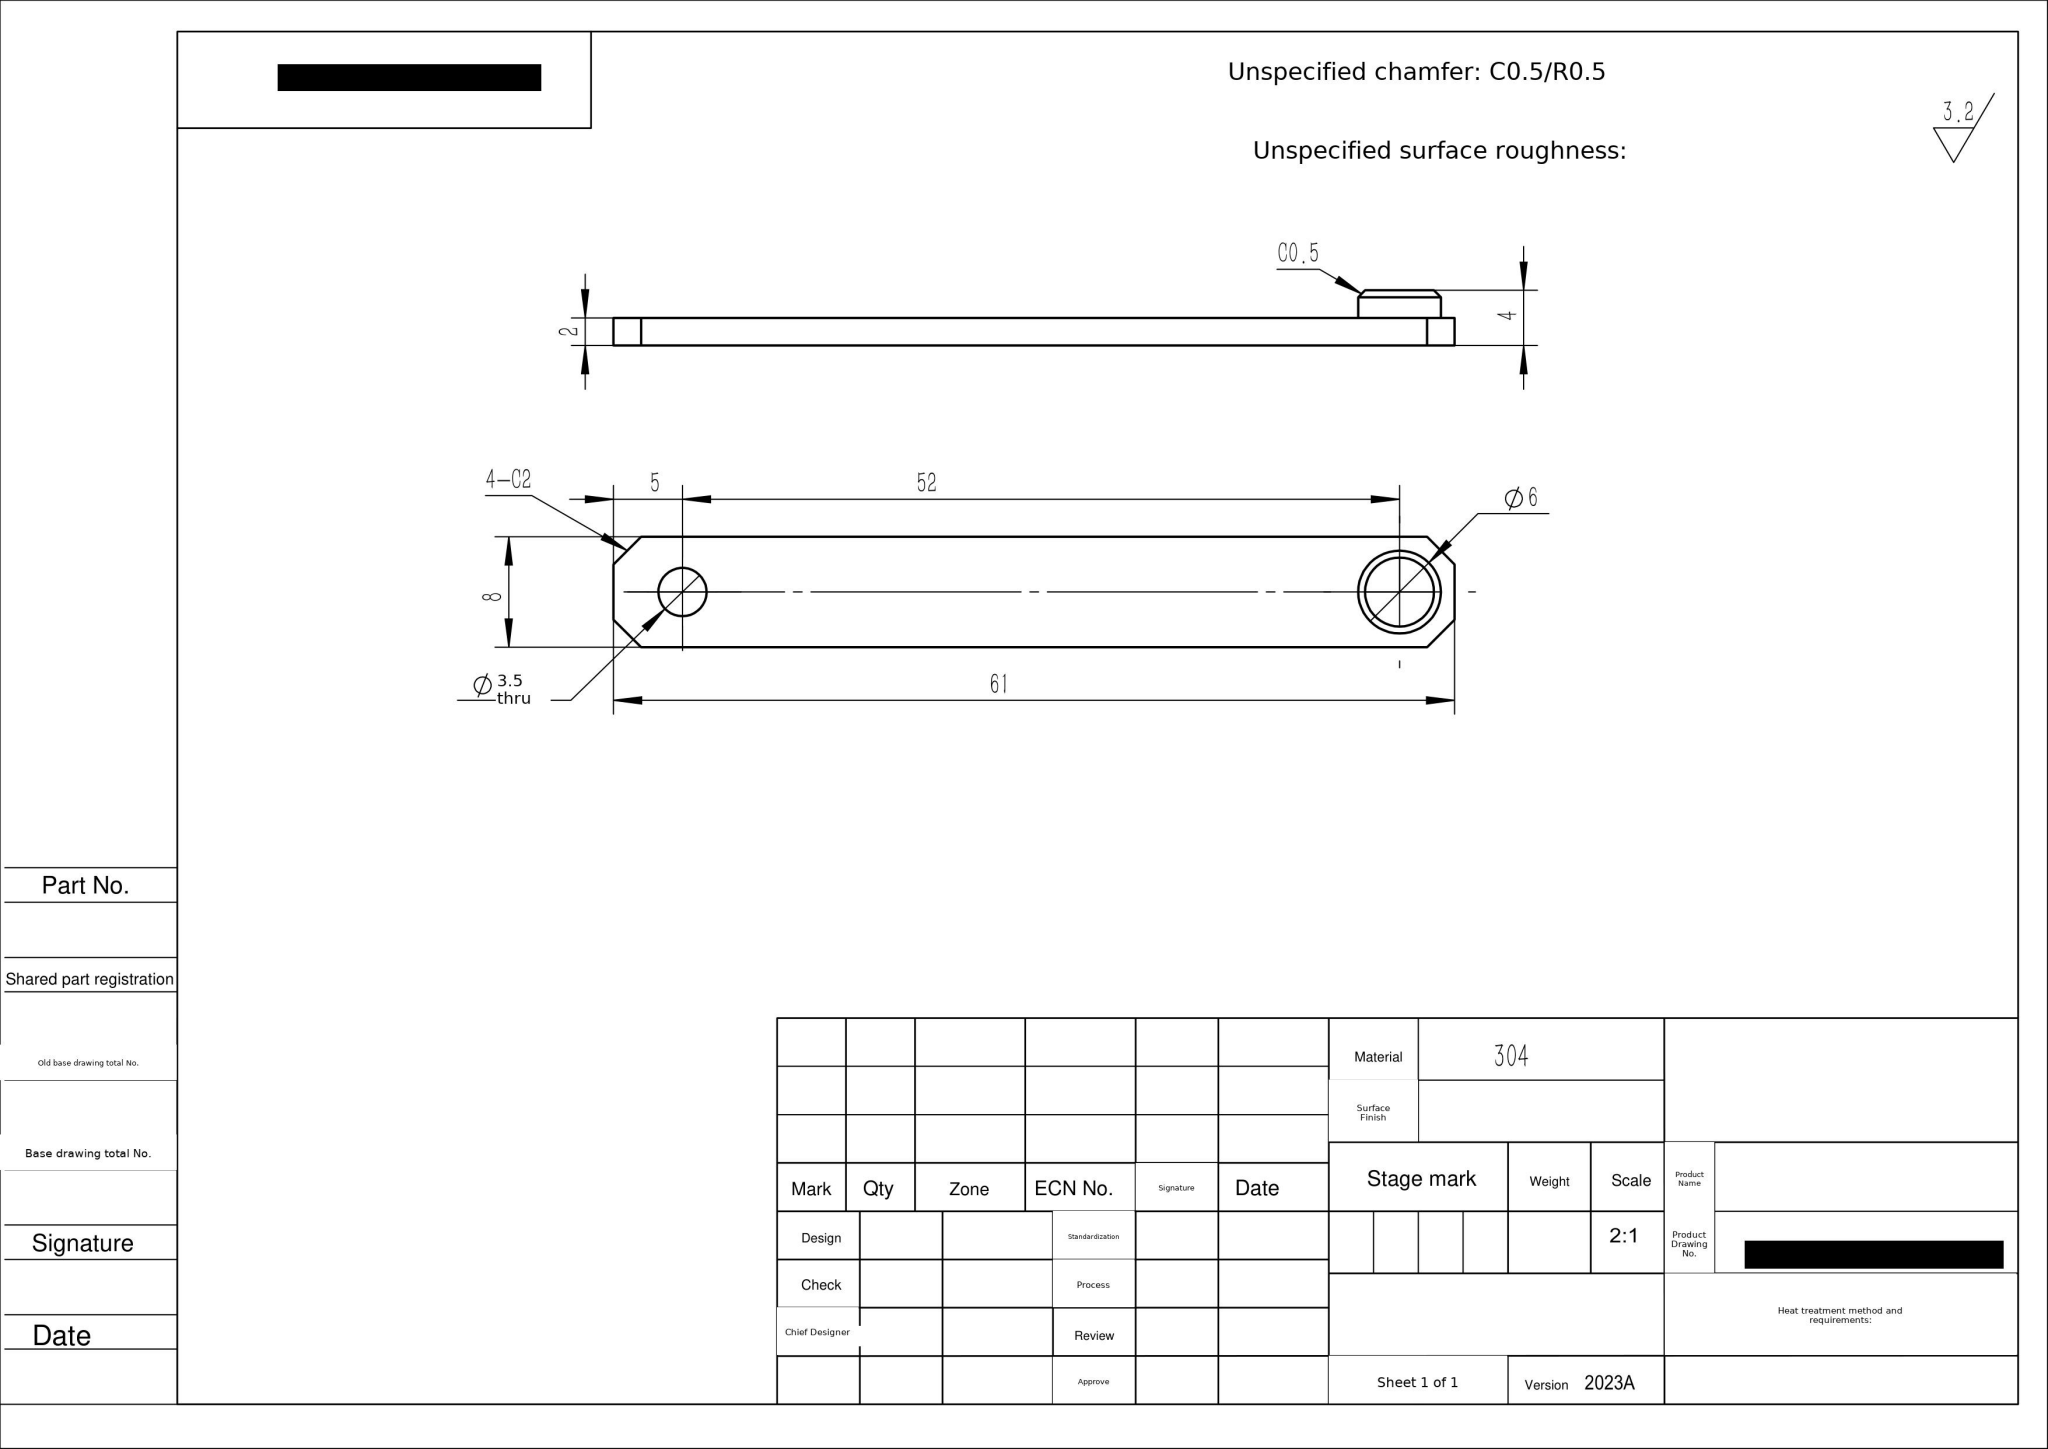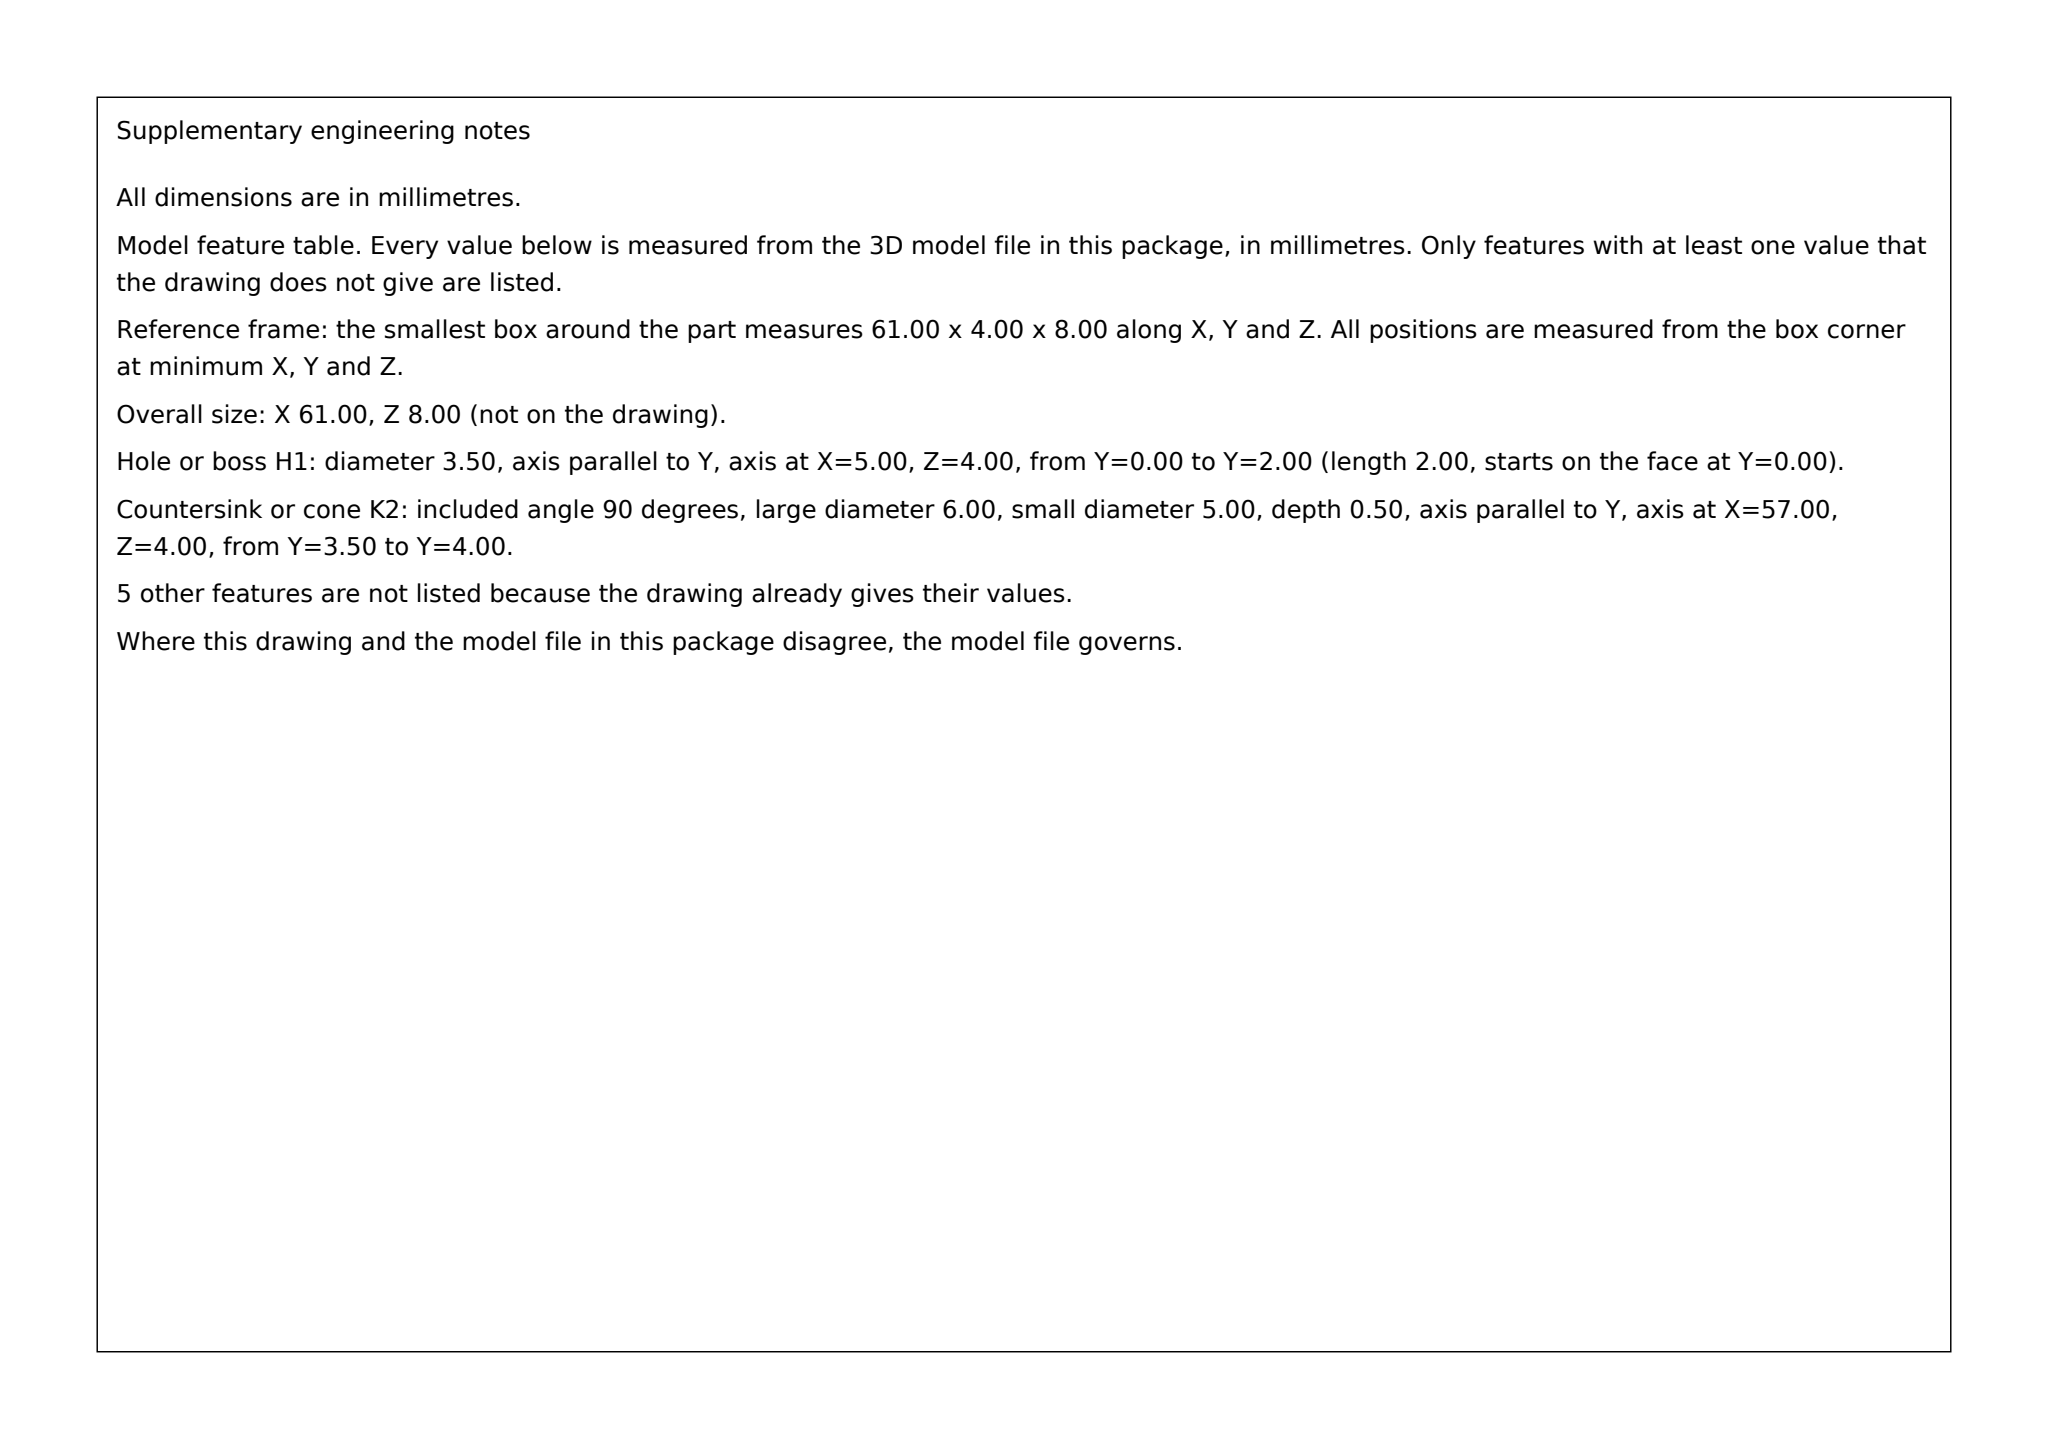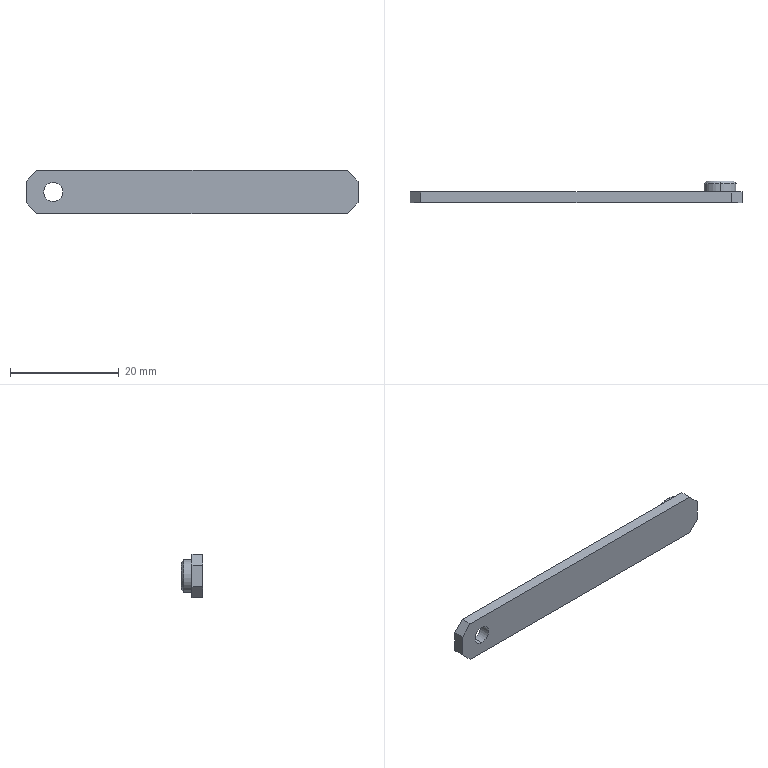Part | SolidWorks | mm | material 304 | 1 solid | 17 faces | box 61 x 4 x 8 mm | volume 995 mm3 | plane 11 | cylinder 4 | cone 2 | commonest cylinder face diameters 6 x2 3.5 x2
build123d program:
from build123d import *

# Parameters (mm, degrees)
SKETCH1_W           = 61
SKETCH1_H           = 8
BOSS_EXTRUDE1_DEPTH = 2
SKETCH2_R           = 1.75
CUT_EXTRUDE1_DEPTH  = 62.555
SKETCH3_R           = 3
BOSS_EXTRUDE2_DEPTH = 2
CHAMFER1_SIZE       = 0.5
CHAMFER2_SIZE       = 2


with BuildPart() as part:
    # Sketch1 → Boss-Extrude1 (new body)
    with BuildSketch(Plane(origin=(0, 0, 0), x_dir=(1, 0, 0), z_dir=(0, 1, 0))):
        with Locations((30.5, 4)):
            Rectangle(SKETCH1_W, SKETCH1_H)
    extrude(amount=BOSS_EXTRUDE1_DEPTH)

    # Sketch2 → Cut-Extrude1 (cut, through all)
    with BuildSketch(Plane(origin=(0, 2, 0), x_dir=(1, 0, 0), z_dir=(0, 1, 0))):
        with Locations(Location((5, 4, 0), (0, 0, 270))):
            Circle(SKETCH2_R)
    extrude(amount=-CUT_EXTRUDE1_DEPTH, mode=Mode.SUBTRACT)

    # Sketch3 → Boss-Extrude2 (add)
    with BuildSketch(Plane(origin=(0, 2, 0), x_dir=(1, 0, 0), z_dir=(0, 1, 0))):
        with Locations(Location((57, 4, 0), (0, 0, 270))):
            Circle(SKETCH3_R)
    extrude(amount=BOSS_EXTRUDE2_DEPTH)

    # Chamfer1
    chamfer1_edges = [part.edges().sort_by_distance(p)[0] for p in [
        (57, 4, -7),
    ]]
    chamfer(chamfer1_edges, length=CHAMFER1_SIZE)

    # Chamfer2
    chamfer2_edges = [part.edges().sort_by_distance(p)[0] for p in [
        (0, 1, -8),
        (61, 1, -8),
        (61, 1, 0),
        (0, 1, 0),
    ]]
    chamfer(chamfer2_edges, length=CHAMFER2_SIZE)


solid = part.part
STEP:
#1=CARTESIAN_POINT('',(57.,4.,-1.5));
#2=VERTEX_POINT('',#1);
#3=CARTESIAN_POINT('',(57.,4.,-6.5));
#4=VERTEX_POINT('',#3);
#5=CARTESIAN_POINT('',(57.,4.,-4.));
#6=DIRECTION('',(0.,1.,0.));
#7=DIRECTION('',(0.,0.,1.));
#8=AXIS2_PLACEMENT_3D('',#5,#6,#7);
#9=CIRCLE('',#8,2.5);
#10=EDGE_CURVE('',#2,#4,#9,.T.);
#11=ORIENTED_EDGE('',*,*,#10,.F.);
#12=CARTESIAN_POINT('',(57.,3.5,-1.));
#13=VERTEX_POINT('',#12);
#14=CARTESIAN_POINT('',(57.,4.,-1.5));
#15=DIRECTION('',(0.,-0.7071,0.7071));
#16=VECTOR('',#15,1000.);
#17=LINE('',#14,#16);
#18=EDGE_CURVE('',#2,#13,#17,.T.);
#19=ORIENTED_EDGE('',*,*,#18,.T.);
#20=CARTESIAN_POINT('',(57.,3.5,-7.));
#21=VERTEX_POINT('',#20);
#22=CARTESIAN_POINT('',(57.,3.5,-4.));
#23=DIRECTION('',(0.,-1.,0.));
#24=DIRECTION('',(0.,0.,1.));
#25=AXIS2_PLACEMENT_3D('',#22,#23,#24);
#26=CIRCLE('',#25,3.);
#27=EDGE_CURVE('',#21,#13,#26,.T.);
#28=ORIENTED_EDGE('',*,*,#27,.F.);
#29=CARTESIAN_POINT('',(57.,4.,-6.5));
#30=DIRECTION('',(0.,-0.7071,-0.7071));
#31=VECTOR('',#30,1000.);
#32=LINE('',#29,#31);
#33=EDGE_CURVE('',#4,#21,#32,.T.);
#34=ORIENTED_EDGE('',*,*,#33,.F.);
#35=EDGE_LOOP('',(#11,#19,#28,#34));
#36=FACE_OUTER_BOUND('',#35,.T.);
#37=CARTESIAN_POINT('',(57.,4.,-4.));
#38=DIRECTION('',(0.,-1.,0.));
#39=DIRECTION('',(0.,0.,-1.));
#40=AXIS2_PLACEMENT_3D('',#37,#38,#39);
#41=CONICAL_SURFACE('',#40,2.5,0.7854);
#42=ADVANCED_FACE('',(#36),#41,.T.);
#43=ORIENTED_EDGE('',*,*,#27,.T.);
#44=CARTESIAN_POINT('',(57.,2.,-1.));
#45=VERTEX_POINT('',#44);
#46=CARTESIAN_POINT('',(57.,4.,-1.));
#47=DIRECTION('',(0.,-1.,0.));
#48=VECTOR('',#47,1000.);
#49=LINE('',#46,#48);
#50=EDGE_CURVE('',#13,#45,#49,.T.);
#51=ORIENTED_EDGE('',*,*,#50,.T.);
#52=CARTESIAN_POINT('',(57.,2.,-7.));
#53=VERTEX_POINT('',#52);
#54=CARTESIAN_POINT('',(57.,2.,-4.));
#55=DIRECTION('',(0.,1.,0.));
#56=DIRECTION('',(0.,0.,1.));
#57=AXIS2_PLACEMENT_3D('',#54,#55,#56);
#58=CIRCLE('',#57,3.);
#59=EDGE_CURVE('',#45,#53,#58,.T.);
#60=ORIENTED_EDGE('',*,*,#59,.T.);
#61=CARTESIAN_POINT('',(57.,4.,-7.));
#62=DIRECTION('',(0.,-1.,0.));
#63=VECTOR('',#62,1000.);
#64=LINE('',#61,#63);
#65=EDGE_CURVE('',#21,#53,#64,.T.);
#66=ORIENTED_EDGE('',*,*,#65,.F.);
#67=EDGE_LOOP('',(#43,#51,#60,#66));
#68=FACE_OUTER_BOUND('',#67,.T.);
#69=CARTESIAN_POINT('',(57.,4.,-4.));
#70=DIRECTION('',(0.,-1.,0.));
#71=DIRECTION('',(0.,0.,-1.));
#72=AXIS2_PLACEMENT_3D('',#69,#70,#71);
#73=CYLINDRICAL_SURFACE('',#72,3.);
#74=ADVANCED_FACE('',(#68),#73,.T.);
#75=CARTESIAN_POINT('',(5.,0.,-5.75));
#76=VERTEX_POINT('',#75);
#77=CARTESIAN_POINT('',(5.,0.,-2.25));
#78=VERTEX_POINT('',#77);
#79=CARTESIAN_POINT('',(5.,0.,-4.));
#80=DIRECTION('',(0.,1.,0.));
#81=DIRECTION('',(0.,0.,1.));
#82=AXIS2_PLACEMENT_3D('',#79,#80,#81);
#83=CIRCLE('',#82,1.75);
#84=EDGE_CURVE('',#76,#78,#83,.T.);
#85=ORIENTED_EDGE('',*,*,#84,.F.);
#86=CARTESIAN_POINT('',(5.,2.,-5.75));
#87=VERTEX_POINT('',#86);
#88=CARTESIAN_POINT('',(5.,0.,-5.75));
#89=DIRECTION('',(0.,1.,0.));
#90=VECTOR('',#89,1000.);
#91=LINE('',#88,#90);
#92=EDGE_CURVE('',#76,#87,#91,.T.);
#93=ORIENTED_EDGE('',*,*,#92,.T.);
#94=CARTESIAN_POINT('',(5.,2.,-2.25));
#95=VERTEX_POINT('',#94);
#96=CARTESIAN_POINT('',(5.,2.,-4.));
#97=DIRECTION('',(0.,1.,0.));
#98=DIRECTION('',(0.,0.,1.));
#99=AXIS2_PLACEMENT_3D('',#96,#97,#98);
#100=CIRCLE('',#99,1.75);
#101=EDGE_CURVE('',#87,#95,#100,.T.);
#102=ORIENTED_EDGE('',*,*,#101,.T.);
#103=CARTESIAN_POINT('',(5.,0.,-2.25));
#104=DIRECTION('',(0.,1.,0.));
#105=VECTOR('',#104,1000.);
#106=LINE('',#103,#105);
#107=EDGE_CURVE('',#78,#95,#106,.T.);
#108=ORIENTED_EDGE('',*,*,#107,.F.);
#109=EDGE_LOOP('',(#85,#93,#102,#108));
#110=FACE_OUTER_BOUND('',#109,.T.);
#111=CARTESIAN_POINT('',(5.,0.,-4.));
#112=DIRECTION('',(0.,1.,0.));
#113=DIRECTION('',(0.,0.,1.));
#114=AXIS2_PLACEMENT_3D('',#111,#112,#113);
#115=CYLINDRICAL_SURFACE('',#114,1.75);
#116=ADVANCED_FACE('',(#110),#115,.F.);
#117=CARTESIAN_POINT('',(61.,2.,-2.));
#118=VERTEX_POINT('',#117);
#119=CARTESIAN_POINT('',(61.,2.,-6.));
#120=VERTEX_POINT('',#119);
#121=CARTESIAN_POINT('',(61.,2.,-8.));
#122=DIRECTION('',(0.,0.,-1.));
#123=VECTOR('',#122,1000.);
#124=LINE('',#121,#123);
#125=EDGE_CURVE('',#118,#120,#124,.T.);
#126=ORIENTED_EDGE('',*,*,#125,.T.);
#127=CARTESIAN_POINT('',(59.,2.,-8.));
#128=VERTEX_POINT('',#127);
#129=CARTESIAN_POINT('',(33.5,2.,-33.5));
#130=DIRECTION('',(-0.7071,0.,-0.7071));
#131=VECTOR('',#130,1000.);
#132=LINE('',#129,#131);
#133=EDGE_CURVE('',#120,#128,#132,.T.);
#134=ORIENTED_EDGE('',*,*,#133,.T.);
#135=CARTESIAN_POINT('',(2.,2.,-8.));
#136=VERTEX_POINT('',#135);
#137=CARTESIAN_POINT('',(0.,2.,-8.));
#138=DIRECTION('',(-1.,0.,0.));
#139=VECTOR('',#138,1000.);
#140=LINE('',#137,#139);
#141=EDGE_CURVE('',#128,#136,#140,.T.);
#142=ORIENTED_EDGE('',*,*,#141,.T.);
#143=CARTESIAN_POINT('',(0.,2.,-6.));
#144=VERTEX_POINT('',#143);
#145=CARTESIAN_POINT('',(-3.,2.,-3.));
#146=DIRECTION('',(-0.7071,0.,0.7071));
#147=VECTOR('',#146,1000.);
#148=LINE('',#145,#147);
#149=EDGE_CURVE('',#136,#144,#148,.T.);
#150=ORIENTED_EDGE('',*,*,#149,.T.);
#151=CARTESIAN_POINT('',(0.,2.,-2.));
#152=VERTEX_POINT('',#151);
#153=CARTESIAN_POINT('',(0.,2.,-8.));
#154=DIRECTION('',(-0.,0.,1.));
#155=VECTOR('',#154,1000.);
#156=LINE('',#153,#155);
#157=EDGE_CURVE('',#144,#152,#156,.T.);
#158=ORIENTED_EDGE('',*,*,#157,.T.);
#159=CARTESIAN_POINT('',(2.,2.,0.));
#160=VERTEX_POINT('',#159);
#161=CARTESIAN_POINT('',(1.,2.,-1.));
#162=DIRECTION('',(0.7071,0.,0.7071));
#163=VECTOR('',#162,1000.);
#164=LINE('',#161,#163);
#165=EDGE_CURVE('',#152,#160,#164,.T.);
#166=ORIENTED_EDGE('',*,*,#165,.T.);
#167=CARTESIAN_POINT('',(59.,2.,0.));
#168=VERTEX_POINT('',#167);
#169=CARTESIAN_POINT('',(0.,2.,0.));
#170=DIRECTION('',(1.,0.,0.));
#171=VECTOR('',#170,1000.);
#172=LINE('',#169,#171);
#173=EDGE_CURVE('',#160,#168,#172,.T.);
#174=ORIENTED_EDGE('',*,*,#173,.T.);
#175=CARTESIAN_POINT('',(29.5,2.,29.5));
#176=DIRECTION('',(0.7071,0.,-0.7071));
#177=VECTOR('',#176,1000.);
#178=LINE('',#175,#177);
#179=EDGE_CURVE('',#168,#118,#178,.T.);
#180=ORIENTED_EDGE('',*,*,#179,.T.);
#181=EDGE_LOOP('',(#126,#134,#142,#150,#158,#166,#174,#180));
#182=FACE_OUTER_BOUND('',#181,.T.);
#183=CARTESIAN_POINT('',(5.,2.,-4.));
#184=DIRECTION('',(0.,1.,0.));
#185=DIRECTION('',(0.,0.,1.));
#186=AXIS2_PLACEMENT_3D('',#183,#184,#185);
#187=CIRCLE('',#186,1.75);
#188=EDGE_CURVE('',#95,#87,#187,.T.);
#189=ORIENTED_EDGE('',*,*,#188,.F.);
#190=ORIENTED_EDGE('',*,*,#101,.F.);
#191=EDGE_LOOP('',(#189,#190));
#192=FACE_BOUND('',#191,.T.);
#193=CARTESIAN_POINT('',(57.,2.,-4.));
#194=DIRECTION('',(0.,1.,0.));
#195=DIRECTION('',(0.,0.,1.));
#196=AXIS2_PLACEMENT_3D('',#193,#194,#195);
#197=CIRCLE('',#196,3.);
#198=EDGE_CURVE('',#53,#45,#197,.T.);
#199=ORIENTED_EDGE('',*,*,#198,.F.);
#200=ORIENTED_EDGE('',*,*,#59,.F.);
#201=EDGE_LOOP('',(#199,#200));
#202=FACE_BOUND('',#201,.T.);
#203=CARTESIAN_POINT('',(0.,2.,0.));
#204=DIRECTION('',(0.,1.,0.));
#205=DIRECTION('',(0.,0.,1.));
#206=AXIS2_PLACEMENT_3D('',#203,#204,#205);
#207=PLANE('',#206);
#208=ADVANCED_FACE('',(#182,#192,#202),#207,.T.);
#209=ORIENTED_EDGE('',*,*,#157,.F.);
#210=CARTESIAN_POINT('',(0.,0.,-6.));
#211=VERTEX_POINT('',#210);
#212=CARTESIAN_POINT('',(0.,2.,-6.));
#213=DIRECTION('',(0.,-1.,0.));
#214=VECTOR('',#213,1000.);
#215=LINE('',#212,#214);
#216=EDGE_CURVE('',#144,#211,#215,.T.);
#217=ORIENTED_EDGE('',*,*,#216,.T.);
#218=CARTESIAN_POINT('',(0.,0.,-2.));
#219=VERTEX_POINT('',#218);
#220=CARTESIAN_POINT('',(0.,0.,-8.));
#221=DIRECTION('',(-0.,0.,1.));
#222=VECTOR('',#221,1000.);
#223=LINE('',#220,#222);
#224=EDGE_CURVE('',#211,#219,#223,.T.);
#225=ORIENTED_EDGE('',*,*,#224,.T.);
#226=CARTESIAN_POINT('',(0.,2.,-2.));
#227=DIRECTION('',(0.,1.,0.));
#228=VECTOR('',#227,1000.);
#229=LINE('',#226,#228);
#230=EDGE_CURVE('',#219,#152,#229,.T.);
#231=ORIENTED_EDGE('',*,*,#230,.T.);
#232=EDGE_LOOP('',(#209,#217,#225,#231));
#233=FACE_OUTER_BOUND('',#232,.T.);
#234=CARTESIAN_POINT('',(0.,2.,-8.));
#235=DIRECTION('',(1.,0.,0.));
#236=DIRECTION('',(0.,0.,-1.));
#237=AXIS2_PLACEMENT_3D('',#234,#235,#236);
#238=PLANE('',#237);
#239=ADVANCED_FACE('',(#233),#238,.F.);
#240=CARTESIAN_POINT('',(2.,0.,0.));
#241=VERTEX_POINT('',#240);
#242=CARTESIAN_POINT('',(59.,0.,0.));
#243=VERTEX_POINT('',#242);
#244=CARTESIAN_POINT('',(0.,0.,0.));
#245=DIRECTION('',(1.,0.,0.));
#246=VECTOR('',#245,1000.);
#247=LINE('',#244,#246);
#248=EDGE_CURVE('',#241,#243,#247,.T.);
#249=ORIENTED_EDGE('',*,*,#248,.T.);
#250=CARTESIAN_POINT('',(59.,2.,0.));
#251=DIRECTION('',(0.,1.,0.));
#252=VECTOR('',#251,1000.);
#253=LINE('',#250,#252);
#254=EDGE_CURVE('',#243,#168,#253,.T.);
#255=ORIENTED_EDGE('',*,*,#254,.T.);
#256=ORIENTED_EDGE('',*,*,#173,.F.);
#257=CARTESIAN_POINT('',(2.,2.,0.));
#258=DIRECTION('',(0.,-1.,0.));
#259=VECTOR('',#258,1000.);
#260=LINE('',#257,#259);
#261=EDGE_CURVE('',#160,#241,#260,.T.);
#262=ORIENTED_EDGE('',*,*,#261,.T.);
#263=EDGE_LOOP('',(#249,#255,#256,#262));
#264=FACE_OUTER_BOUND('',#263,.T.);
#265=CARTESIAN_POINT('',(0.,2.,0.));
#266=DIRECTION('',(0.,0.,-1.));
#267=DIRECTION('',(-1.,0.,0.));
#268=AXIS2_PLACEMENT_3D('',#265,#266,#267);
#269=PLANE('',#268);
#270=ADVANCED_FACE('',(#264),#269,.F.);
#271=CARTESIAN_POINT('',(61.,0.,-2.));
#272=VERTEX_POINT('',#271);
#273=CARTESIAN_POINT('',(61.,0.,-6.));
#274=VERTEX_POINT('',#273);
#275=CARTESIAN_POINT('',(61.,0.,-8.));
#276=DIRECTION('',(0.,0.,-1.));
#277=VECTOR('',#276,1000.);
#278=LINE('',#275,#277);
#279=EDGE_CURVE('',#272,#274,#278,.T.);
#280=ORIENTED_EDGE('',*,*,#279,.T.);
#281=CARTESIAN_POINT('',(61.,2.,-6.));
#282=DIRECTION('',(0.,1.,0.));
#283=VECTOR('',#282,1000.);
#284=LINE('',#281,#283);
#285=EDGE_CURVE('',#274,#120,#284,.T.);
#286=ORIENTED_EDGE('',*,*,#285,.T.);
#287=ORIENTED_EDGE('',*,*,#125,.F.);
#288=CARTESIAN_POINT('',(61.,2.,-2.));
#289=DIRECTION('',(0.,-1.,0.));
#290=VECTOR('',#289,1000.);
#291=LINE('',#288,#290);
#292=EDGE_CURVE('',#118,#272,#291,.T.);
#293=ORIENTED_EDGE('',*,*,#292,.T.);
#294=EDGE_LOOP('',(#280,#286,#287,#293));
#295=FACE_OUTER_BOUND('',#294,.T.);
#296=CARTESIAN_POINT('',(61.,2.,-8.));
#297=DIRECTION('',(-1.,0.,0.));
#298=DIRECTION('',(0.,0.,1.));
#299=AXIS2_PLACEMENT_3D('',#296,#297,#298);
#300=PLANE('',#299);
#301=ADVANCED_FACE('',(#295),#300,.F.);
#302=ORIENTED_EDGE('',*,*,#141,.F.);
#303=CARTESIAN_POINT('',(59.,0.,-8.));
#304=VERTEX_POINT('',#303);
#305=CARTESIAN_POINT('',(59.,2.,-8.));
#306=DIRECTION('',(0.,-1.,0.));
#307=VECTOR('',#306,1000.);
#308=LINE('',#305,#307);
#309=EDGE_CURVE('',#128,#304,#308,.T.);
#310=ORIENTED_EDGE('',*,*,#309,.T.);
#311=CARTESIAN_POINT('',(2.,0.,-8.));
#312=VERTEX_POINT('',#311);
#313=CARTESIAN_POINT('',(0.,0.,-8.));
#314=DIRECTION('',(-1.,0.,0.));
#315=VECTOR('',#314,1000.);
#316=LINE('',#313,#315);
#317=EDGE_CURVE('',#304,#312,#316,.T.);
#318=ORIENTED_EDGE('',*,*,#317,.T.);
#319=CARTESIAN_POINT('',(2.,2.,-8.));
#320=DIRECTION('',(0.,1.,0.));
#321=VECTOR('',#320,1000.);
#322=LINE('',#319,#321);
#323=EDGE_CURVE('',#312,#136,#322,.T.);
#324=ORIENTED_EDGE('',*,*,#323,.T.);
#325=EDGE_LOOP('',(#302,#310,#318,#324));
#326=FACE_OUTER_BOUND('',#325,.T.);
#327=CARTESIAN_POINT('',(0.,2.,-8.));
#328=DIRECTION('',(0.,0.,1.));
#329=DIRECTION('',(1.,0.,0.));
#330=AXIS2_PLACEMENT_3D('',#327,#328,#329);
#331=PLANE('',#330);
#332=ADVANCED_FACE('',(#326),#331,.F.);
#333=CARTESIAN_POINT('',(5.,0.,-4.));
#334=DIRECTION('',(0.,1.,0.));
#335=DIRECTION('',(0.,0.,1.));
#336=AXIS2_PLACEMENT_3D('',#333,#334,#335);
#337=CIRCLE('',#336,1.75);
#338=EDGE_CURVE('',#78,#76,#337,.T.);
#339=ORIENTED_EDGE('',*,*,#338,.T.);
#340=ORIENTED_EDGE('',*,*,#84,.T.);
#341=EDGE_LOOP('',(#339,#340));
#342=FACE_BOUND('',#341,.T.);
#343=ORIENTED_EDGE('',*,*,#317,.F.);
#344=CARTESIAN_POINT('',(59.,0.,-8.));
#345=DIRECTION('',(0.7071,0.,0.7071));
#346=VECTOR('',#345,1000.);
#347=LINE('',#344,#346);
#348=EDGE_CURVE('',#304,#274,#347,.T.);
#349=ORIENTED_EDGE('',*,*,#348,.T.);
#350=ORIENTED_EDGE('',*,*,#279,.F.);
#351=CARTESIAN_POINT('',(61.,0.,-2.));
#352=DIRECTION('',(-0.7071,0.,0.7071));
#353=VECTOR('',#352,1000.);
#354=LINE('',#351,#353);
#355=EDGE_CURVE('',#272,#243,#354,.T.);
#356=ORIENTED_EDGE('',*,*,#355,.T.);
#357=ORIENTED_EDGE('',*,*,#248,.F.);
#358=CARTESIAN_POINT('',(2.,0.,0.));
#359=DIRECTION('',(-0.7071,0.,-0.7071));
#360=VECTOR('',#359,1000.);
#361=LINE('',#358,#360);
#362=EDGE_CURVE('',#241,#219,#361,.T.);
#363=ORIENTED_EDGE('',*,*,#362,.T.);
#364=ORIENTED_EDGE('',*,*,#224,.F.);
#365=CARTESIAN_POINT('',(0.,0.,-6.));
#366=DIRECTION('',(0.7071,0.,-0.7071));
#367=VECTOR('',#366,1000.);
#368=LINE('',#365,#367);
#369=EDGE_CURVE('',#211,#312,#368,.T.);
#370=ORIENTED_EDGE('',*,*,#369,.T.);
#371=EDGE_LOOP('',(#343,#349,#350,#356,#357,#363,#364,#370));
#372=FACE_OUTER_BOUND('',#371,.T.);
#373=CARTESIAN_POINT('',(0.,0.,0.));
#374=DIRECTION('',(0.,1.,0.));
#375=DIRECTION('',(0.,0.,1.));
#376=AXIS2_PLACEMENT_3D('',#373,#374,#375);
#377=PLANE('',#376);
#378=ADVANCED_FACE('',(#342,#372),#377,.F.);
#379=ORIENTED_EDGE('',*,*,#92,.F.);
#380=ORIENTED_EDGE('',*,*,#338,.F.);
#381=ORIENTED_EDGE('',*,*,#107,.T.);
#382=ORIENTED_EDGE('',*,*,#188,.T.);
#383=EDGE_LOOP('',(#379,#380,#381,#382));
#384=FACE_OUTER_BOUND('',#383,.T.);
#385=CARTESIAN_POINT('',(5.,0.,-4.));
#386=DIRECTION('',(0.,1.,0.));
#387=DIRECTION('',(0.,0.,1.));
#388=AXIS2_PLACEMENT_3D('',#385,#386,#387);
#389=CYLINDRICAL_SURFACE('',#388,1.75);
#390=ADVANCED_FACE('',(#384),#389,.F.);
#391=ORIENTED_EDGE('',*,*,#50,.F.);
#392=CARTESIAN_POINT('',(57.,3.5,-4.));
#393=DIRECTION('',(0.,-1.,0.));
#394=DIRECTION('',(0.,0.,1.));
#395=AXIS2_PLACEMENT_3D('',#392,#393,#394);
#396=CIRCLE('',#395,3.);
#397=EDGE_CURVE('',#13,#21,#396,.T.);
#398=ORIENTED_EDGE('',*,*,#397,.T.);
#399=ORIENTED_EDGE('',*,*,#65,.T.);
#400=ORIENTED_EDGE('',*,*,#198,.T.);
#401=EDGE_LOOP('',(#391,#398,#399,#400));
#402=FACE_OUTER_BOUND('',#401,.T.);
#403=CARTESIAN_POINT('',(57.,4.,-4.));
#404=DIRECTION('',(0.,-1.,0.));
#405=DIRECTION('',(0.,0.,-1.));
#406=AXIS2_PLACEMENT_3D('',#403,#404,#405);
#407=CYLINDRICAL_SURFACE('',#406,3.);
#408=ADVANCED_FACE('',(#402),#407,.T.);
#409=CARTESIAN_POINT('',(57.,4.,-4.));
#410=DIRECTION('',(0.,1.,0.));
#411=DIRECTION('',(0.,0.,1.));
#412=AXIS2_PLACEMENT_3D('',#409,#410,#411);
#413=CIRCLE('',#412,2.5);
#414=EDGE_CURVE('',#4,#2,#413,.T.);
#415=ORIENTED_EDGE('',*,*,#414,.T.);
#416=ORIENTED_EDGE('',*,*,#10,.T.);
#417=EDGE_LOOP('',(#415,#416));
#418=FACE_OUTER_BOUND('',#417,.T.);
#419=CARTESIAN_POINT('',(57.,4.,-4.));
#420=DIRECTION('',(0.,1.,0.));
#421=DIRECTION('',(0.,0.,1.));
#422=AXIS2_PLACEMENT_3D('',#419,#420,#421);
#423=PLANE('',#422);
#424=ADVANCED_FACE('',(#418),#423,.T.);
#425=ORIENTED_EDGE('',*,*,#18,.F.);
#426=ORIENTED_EDGE('',*,*,#414,.F.);
#427=ORIENTED_EDGE('',*,*,#33,.T.);
#428=ORIENTED_EDGE('',*,*,#397,.F.);
#429=EDGE_LOOP('',(#425,#426,#427,#428));
#430=FACE_OUTER_BOUND('',#429,.T.);
#431=CARTESIAN_POINT('',(57.,4.,-4.));
#432=DIRECTION('',(0.,-1.,0.));
#433=DIRECTION('',(0.,0.,-1.));
#434=AXIS2_PLACEMENT_3D('',#431,#432,#433);
#435=CONICAL_SURFACE('',#434,2.5,0.7854);
#436=ADVANCED_FACE('',(#430),#435,.T.);
#437=ORIENTED_EDGE('',*,*,#133,.F.);
#438=ORIENTED_EDGE('',*,*,#285,.F.);
#439=ORIENTED_EDGE('',*,*,#348,.F.);
#440=ORIENTED_EDGE('',*,*,#309,.F.);
#441=EDGE_LOOP('',(#437,#438,#439,#440));
#442=FACE_OUTER_BOUND('',#441,.T.);
#443=CARTESIAN_POINT('',(59.,2.,-8.));
#444=DIRECTION('',(-0.7071,0.,0.7071));
#445=DIRECTION('',(0.,-1.,0.));
#446=AXIS2_PLACEMENT_3D('',#443,#444,#445);
#447=PLANE('',#446);
#448=ADVANCED_FACE('',(#442),#447,.F.);
#449=ORIENTED_EDGE('',*,*,#179,.F.);
#450=ORIENTED_EDGE('',*,*,#254,.F.);
#451=ORIENTED_EDGE('',*,*,#355,.F.);
#452=ORIENTED_EDGE('',*,*,#292,.F.);
#453=EDGE_LOOP('',(#449,#450,#451,#452));
#454=FACE_OUTER_BOUND('',#453,.T.);
#455=CARTESIAN_POINT('',(61.,2.,-2.));
#456=DIRECTION('',(-0.7071,0.,-0.7071));
#457=DIRECTION('',(0.,-1.,0.));
#458=AXIS2_PLACEMENT_3D('',#455,#456,#457);
#459=PLANE('',#458);
#460=ADVANCED_FACE('',(#454),#459,.F.);
#461=ORIENTED_EDGE('',*,*,#149,.F.);
#462=ORIENTED_EDGE('',*,*,#323,.F.);
#463=ORIENTED_EDGE('',*,*,#369,.F.);
#464=ORIENTED_EDGE('',*,*,#216,.F.);
#465=EDGE_LOOP('',(#461,#462,#463,#464));
#466=FACE_OUTER_BOUND('',#465,.T.);
#467=CARTESIAN_POINT('',(0.,2.,-6.));
#468=DIRECTION('',(0.7071,0.,0.7071));
#469=DIRECTION('',(0.,-1.,0.));
#470=AXIS2_PLACEMENT_3D('',#467,#468,#469);
#471=PLANE('',#470);
#472=ADVANCED_FACE('',(#466),#471,.F.);
#473=ORIENTED_EDGE('',*,*,#165,.F.);
#474=ORIENTED_EDGE('',*,*,#230,.F.);
#475=ORIENTED_EDGE('',*,*,#362,.F.);
#476=ORIENTED_EDGE('',*,*,#261,.F.);
#477=EDGE_LOOP('',(#473,#474,#475,#476));
#478=FACE_OUTER_BOUND('',#477,.T.);
#479=CARTESIAN_POINT('',(2.,2.,0.));
#480=DIRECTION('',(0.7071,0.,-0.7071));
#481=DIRECTION('',(0.,-1.,0.));
#482=AXIS2_PLACEMENT_3D('',#479,#480,#481);
#483=PLANE('',#482);
#484=ADVANCED_FACE('',(#478),#483,.F.);
#485=CLOSED_SHELL('',(#42,#74,#116,#208,#239,#270,#301,#332,#378,#390,#408,#424,#436,#448,#460,#472,#484));
#486=MANIFOLD_SOLID_BREP('',#485);
#487=CARTESIAN_POINT('',(0.,0.,0.));
#488=DIRECTION('',(0.,0.,1.));
#489=DIRECTION('',(1.,0.,0.));
#490=AXIS2_PLACEMENT_3D('',#487,#488,#489);
#491=(LENGTH_UNIT()NAMED_UNIT(*)SI_UNIT(.MILLI.,.METRE.));
#492=UNCERTAINTY_MEASURE_WITH_UNIT(LENGTH_MEASURE(0.00001),#491,'','');
#493=(NAMED_UNIT(*)PLANE_ANGLE_UNIT()SI_UNIT($,.RADIAN.));
#494=(NAMED_UNIT(*)SI_UNIT($,.STERADIAN.)SOLID_ANGLE_UNIT());
#495=(GEOMETRIC_REPRESENTATION_CONTEXT(3)GLOBAL_UNCERTAINTY_ASSIGNED_CONTEXT((#492))GLOBAL_UNIT_ASSIGNED_CONTEXT((#491,#493,#494))REPRESENTATION_CONTEXT('',''));
#496=ADVANCED_BREP_SHAPE_REPRESENTATION('',(#486,#490),#495);